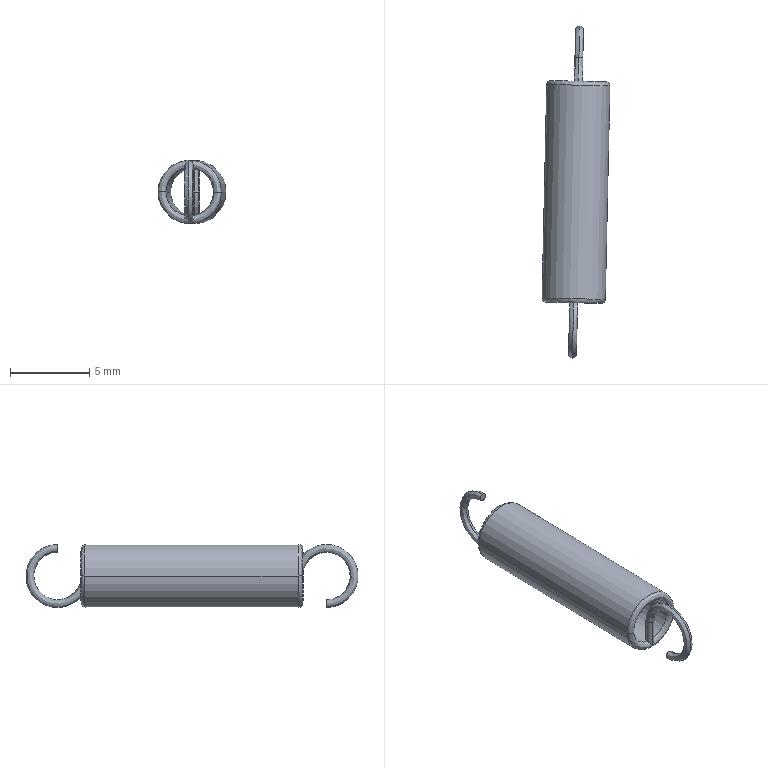Component | SolidWorks | YAUS-D4-L20-1 | 1 solid | 18 faces | box 4.29 x 21 x 4 mm | volume 80 mm3 | spline 8 | cylinder 8 | plane 2 | commonest cylinder face diameters 0.5 x4 4 x2 3 x2
STEP:
#1=CARTESIAN_POINT('',(-2.297,-0.5365,1.426));
#2=VERTEX_POINT('',#1);
#3=CARTESIAN_POINT('',(-2.347,-0.5355,1.485));
#4=VERTEX_POINT('',#3);
#5=CARTESIAN_POINT('',(-2.287,-0.5368,1.485));
#6=DIRECTION('',(0.0216,0.9998,-0.));
#7=DIRECTION('',(0.9998,-0.0216,0.));
#8=AXIS2_PLACEMENT_3D('',#5,#6,#7);
#9=CIRCLE('',#8,0.05906);
#10=EDGE_CURVE('',#2,#4,#9,.T.);
#11=ORIENTED_EDGE('',*,*,#10,.T.);
#12=CARTESIAN_POINT('',(-2.366,-0.5351,1.485));
#13=VERTEX_POINT('',#12);
#14=CARTESIAN_POINT('',(-2.356,-0.5353,1.485));
#15=DIRECTION('',(-0.,0.,-1.));
#16=DIRECTION('',(-0.9998,0.0216,0.));
#17=AXIS2_PLACEMENT_3D('',#14,#15,#16);
#18=CIRCLE('',#17,0.009843);
#19=EDGE_CURVE('',#4,#13,#18,.T.);
#20=ORIENTED_EDGE('',*,*,#19,.T.);
#21=CARTESIAN_POINT('',(-2.209,-0.5385,1.485));
#22=VERTEX_POINT('',#21);
#23=CARTESIAN_POINT('',(-2.287,-0.5368,1.485));
#24=DIRECTION('',(0.0216,0.9998,-0.));
#25=DIRECTION('',(-0.9998,0.0216,0.));
#26=AXIS2_PLACEMENT_3D('',#23,#24,#25);
#27=CIRCLE('',#26,0.07874);
#28=EDGE_CURVE('',#22,#13,#27,.T.);
#29=ORIENTED_EDGE('',*,*,#28,.F.);
#30=CARTESIAN_POINT('',(-2.228,-0.538,1.485));
#31=VERTEX_POINT('',#30);
#32=CARTESIAN_POINT('',(-2.219,-0.5382,1.485));
#33=DIRECTION('',(0.,0.,1.));
#34=DIRECTION('',(0.9998,-0.0216,0.));
#35=AXIS2_PLACEMENT_3D('',#32,#33,#34);
#36=CIRCLE('',#35,0.009843);
#37=EDGE_CURVE('',#31,#22,#36,.T.);
#38=ORIENTED_EDGE('',*,*,#37,.F.);
#39=CARTESIAN_POINT('',(-2.278,-0.537,1.426));
#40=VERTEX_POINT('',#39);
#41=CARTESIAN_POINT('',(-2.287,-0.5368,1.485));
#42=DIRECTION('',(0.0216,0.9998,-0.));
#43=DIRECTION('',(0.9998,-0.0216,0.));
#44=AXIS2_PLACEMENT_3D('',#41,#42,#43);
#45=CIRCLE('',#44,0.05906);
#46=EDGE_CURVE('',#31,#40,#45,.T.);
#47=ORIENTED_EDGE('',*,*,#46,.T.);
#48=CARTESIAN_POINT('',(-2.288,-0.5466,1.416));
#49=VERTEX_POINT('',#48);
#50=CARTESIAN_POINT('',(-2.278,-0.537,1.426));
#51=CARTESIAN_POINT('',(-2.278,-0.5377,1.426));
#52=CARTESIAN_POINT('',(-2.278,-0.5385,1.426));
#53=CARTESIAN_POINT('',(-2.278,-0.5396,1.426));
#54=CARTESIAN_POINT('',(-2.278,-0.5401,1.426));
#55=CARTESIAN_POINT('',(-2.278,-0.5407,1.425));
#56=CARTESIAN_POINT('',(-2.279,-0.541,1.425));
#57=CARTESIAN_POINT('',(-2.279,-0.5413,1.425));
#58=CARTESIAN_POINT('',(-2.279,-0.5419,1.425));
#59=CARTESIAN_POINT('',(-2.279,-0.5424,1.424));
#60=CARTESIAN_POINT('',(-2.28,-0.5432,1.424));
#61=CARTESIAN_POINT('',(-2.28,-0.5436,1.423));
#62=CARTESIAN_POINT('',(-2.281,-0.544,1.423));
#63=CARTESIAN_POINT('',(-2.281,-0.5442,1.423));
#64=CARTESIAN_POINT('',(-2.281,-0.5443,1.422));
#65=CARTESIAN_POINT('',(-2.281,-0.5444,1.422));
#66=CARTESIAN_POINT('',(-2.282,-0.5447,1.422));
#67=CARTESIAN_POINT('',(-2.282,-0.545,1.422));
#68=CARTESIAN_POINT('',(-2.283,-0.5454,1.421));
#69=CARTESIAN_POINT('',(-2.283,-0.5456,1.42));
#70=CARTESIAN_POINT('',(-2.284,-0.5459,1.42));
#71=CARTESIAN_POINT('',(-2.284,-0.546,1.419));
#72=CARTESIAN_POINT('',(-2.286,-0.5466,1.417));
#73=CARTESIAN_POINT('',(-2.287,-0.5466,1.416));
#74=CARTESIAN_POINT('',(-2.288,-0.5466,1.416));
#75=B_SPLINE_CURVE_WITH_KNOTS('',3,(#50,#51,#52,#53,#54,#55,#56,#57,#58,#59,#60,#61,#62,#63,#64,#65,#66,#67,#68,#69,#70,#71,#72,#73,#74),.UNSPECIFIED.,.F.,.F.,(4,2,1,2,2,2,1,1,2,2,2,2,2,4),(0.,0.125,0.1875,0.2187,0.25,0.375,0.4375,0.4687,0.4844,0.5,0.625,0.6875,0.75,1.),.UNSPECIFIED.);
#76=EDGE_CURVE('',#40,#49,#75,.T.);
#77=ORIENTED_EDGE('',*,*,#76,.T.);
#78=CARTESIAN_POINT('',(-2.288,-0.5466,1.416));
#79=CARTESIAN_POINT('',(-2.288,-0.5466,1.416));
#80=CARTESIAN_POINT('',(-2.288,-0.5466,1.416));
#81=CARTESIAN_POINT('',(-2.289,-0.5464,1.417));
#82=CARTESIAN_POINT('',(-2.29,-0.5464,1.418));
#83=CARTESIAN_POINT('',(-2.29,-0.5462,1.418));
#84=CARTESIAN_POINT('',(-2.291,-0.5461,1.419));
#85=CARTESIAN_POINT('',(-2.292,-0.5457,1.42));
#86=CARTESIAN_POINT('',(-2.292,-0.5454,1.42));
#87=CARTESIAN_POINT('',(-2.293,-0.5449,1.421));
#88=CARTESIAN_POINT('',(-2.293,-0.5448,1.421));
#89=CARTESIAN_POINT('',(-2.294,-0.5445,1.422));
#90=CARTESIAN_POINT('',(-2.294,-0.5444,1.422));
#91=CARTESIAN_POINT('',(-2.294,-0.5443,1.422));
#92=CARTESIAN_POINT('',(-2.294,-0.5442,1.422));
#93=CARTESIAN_POINT('',(-2.294,-0.5442,1.422));
#94=CARTESIAN_POINT('',(-2.295,-0.5437,1.423));
#95=CARTESIAN_POINT('',(-2.295,-0.5431,1.423));
#96=CARTESIAN_POINT('',(-2.296,-0.5424,1.424));
#97=CARTESIAN_POINT('',(-2.296,-0.542,1.424));
#98=CARTESIAN_POINT('',(-2.296,-0.5416,1.425));
#99=CARTESIAN_POINT('',(-2.296,-0.5413,1.425));
#100=CARTESIAN_POINT('',(-2.296,-0.5412,1.425));
#101=CARTESIAN_POINT('',(-2.297,-0.5396,1.426));
#102=CARTESIAN_POINT('',(-2.297,-0.538,1.426));
#103=CARTESIAN_POINT('',(-2.297,-0.5365,1.426));
#104=B_SPLINE_CURVE_WITH_KNOTS('',3,(#78,#79,#80,#81,#82,#83,#84,#85,#86,#87,#88,#89,#90,#91,#92,#93,#94,#95,#96,#97,#98,#99,#100,#101,#102,#103),.UNSPECIFIED.,.F.,.F.,(4,2,2,2,2,2,1,2,2,2,1,2,2,4),(0.,0.125,0.1875,0.25,0.375,0.4375,0.4688,0.4844,0.5,0.625,0.6875,0.7188,0.75,1.),.UNSPECIFIED.);
#105=EDGE_CURVE('',#49,#2,#104,.T.);
#106=ORIENTED_EDGE('',*,*,#105,.T.);
#107=EDGE_LOOP('',(#11,#20,#29,#38,#47,#77,#106));
#108=FACE_OUTER_BOUND('',#107,.T.);
#109=CARTESIAN_POINT('',(-2.347,-0.5355,1.485));
#110=CARTESIAN_POINT('',(-2.347,-0.5355,1.366));
#111=CARTESIAN_POINT('',(-2.228,-0.538,1.366));
#112=CARTESIAN_POINT('',(-2.228,-0.538,1.485));
#113=CARTESIAN_POINT('',(-2.347,-0.5412,1.485));
#114=CARTESIAN_POINT('',(-2.347,-0.5412,1.366));
#115=CARTESIAN_POINT('',(-2.229,-0.5438,1.366));
#116=CARTESIAN_POINT('',(-2.229,-0.5438,1.485));
#117=CARTESIAN_POINT('',(-2.351,-0.5452,1.485));
#118=CARTESIAN_POINT('',(-2.351,-0.5452,1.358));
#119=CARTESIAN_POINT('',(-2.225,-0.548,1.358));
#120=CARTESIAN_POINT('',(-2.225,-0.548,1.485));
#121=CARTESIAN_POINT('',(-2.357,-0.5451,1.485));
#122=CARTESIAN_POINT('',(-2.357,-0.5451,1.347));
#123=CARTESIAN_POINT('',(-2.219,-0.5481,1.347));
#124=CARTESIAN_POINT('',(-2.219,-0.5481,1.485));
#125=CARTESIAN_POINT('',(-2.362,-0.545,1.485));
#126=CARTESIAN_POINT('',(-2.362,-0.545,1.335));
#127=CARTESIAN_POINT('',(-2.213,-0.5482,1.335));
#128=CARTESIAN_POINT('',(-2.213,-0.5482,1.485));
#129=CARTESIAN_POINT('',(-2.366,-0.5408,1.485));
#130=CARTESIAN_POINT('',(-2.366,-0.5408,1.327));
#131=CARTESIAN_POINT('',(-2.209,-0.5442,1.327));
#132=CARTESIAN_POINT('',(-2.209,-0.5442,1.485));
#133=CARTESIAN_POINT('',(-2.366,-0.5351,1.485));
#134=CARTESIAN_POINT('',(-2.366,-0.5351,1.327));
#135=CARTESIAN_POINT('',(-2.209,-0.5385,1.327));
#136=CARTESIAN_POINT('',(-2.209,-0.5385,1.485));
#137=(BOUNDED_SURFACE()B_SPLINE_SURFACE(3,3,((#109,#110,#111,#112),(#113,#114,#115,#116),(#117,#118,#119,#120),(#121,#122,#123,#124),(#125,#126,#127,#128),(#129,#130,#131,#132),(#133,#134,#135,#136)),.UNSPECIFIED.,.F.,.F.,.F.)B_SPLINE_SURFACE_WITH_KNOTS((4,3,4),(4,4),(0.,0.5,1.),(0.,1.),.UNSPECIFIED.)GEOMETRIC_REPRESENTATION_ITEM()RATIONAL_B_SPLINE_SURFACE(((1.,0.3333,0.3333,1.),(0.8047,0.2682,0.2682,0.8047),(0.8047,0.2682,0.2682,0.8047),(1.,0.3333,0.3333,1.),(0.8047,0.2682,0.2682,0.8047),(0.8047,0.2682,0.2682,0.8047),(1.,0.3333,0.3333,1.)))REPRESENTATION_ITEM('')SURFACE());
#138=ADVANCED_FACE('',(#108),#137,.T.);
#139=CARTESIAN_POINT('',(-2.355,-0.003688,1.485));
#140=VERTEX_POINT('',#139);
#141=CARTESIAN_POINT('',(-2.197,-0.007089,1.485));
#142=VERTEX_POINT('',#141);
#143=CARTESIAN_POINT('',(-2.276,-0.005388,1.485));
#144=DIRECTION('',(-0.0216,-0.9998,0.));
#145=DIRECTION('',(-0.9998,0.0216,0.));
#146=AXIS2_PLACEMENT_3D('',#143,#144,#145);
#147=CIRCLE('',#146,0.07874);
#148=EDGE_CURVE('',#140,#142,#147,.T.);
#149=ORIENTED_EDGE('',*,*,#148,.F.);
#150=CARTESIAN_POINT('',(-2.335,-0.004113,1.485));
#151=VERTEX_POINT('',#150);
#152=CARTESIAN_POINT('',(-2.345,-0.003901,1.485));
#153=DIRECTION('',(-0.,0.,-1.));
#154=DIRECTION('',(-0.9998,0.0216,0.));
#155=AXIS2_PLACEMENT_3D('',#152,#153,#154);
#156=CIRCLE('',#155,0.009843);
#157=EDGE_CURVE('',#140,#151,#156,.T.);
#158=ORIENTED_EDGE('',*,*,#157,.T.);
#159=CARTESIAN_POINT('',(-2.217,-0.006664,1.485));
#160=VERTEX_POINT('',#159);
#161=CARTESIAN_POINT('',(-2.276,-0.005388,1.485));
#162=DIRECTION('',(-0.0216,-0.9998,0.));
#163=DIRECTION('',(0.9998,-0.0216,0.));
#164=AXIS2_PLACEMENT_3D('',#161,#162,#163);
#165=CIRCLE('',#164,0.05906);
#166=EDGE_CURVE('',#151,#160,#165,.T.);
#167=ORIENTED_EDGE('',*,*,#166,.T.);
#168=CARTESIAN_POINT('',(-2.207,-0.006876,1.485));
#169=DIRECTION('',(0.,0.,1.));
#170=DIRECTION('',(0.9998,-0.0216,0.));
#171=AXIS2_PLACEMENT_3D('',#168,#169,#170);
#172=CIRCLE('',#171,0.009843);
#173=EDGE_CURVE('',#142,#160,#172,.T.);
#174=ORIENTED_EDGE('',*,*,#173,.F.);
#175=EDGE_LOOP('',(#149,#158,#167,#174));
#176=FACE_OUTER_BOUND('',#175,.T.);
#177=CARTESIAN_POINT('',(-2.355,-0.003688,1.485));
#178=CARTESIAN_POINT('',(-2.355,-0.003688,1.327));
#179=CARTESIAN_POINT('',(-2.197,-0.007089,1.327));
#180=CARTESIAN_POINT('',(-2.197,-0.007089,1.485));
#181=CARTESIAN_POINT('',(-2.354,0.01599,1.485));
#182=CARTESIAN_POINT('',(-2.354,0.01599,1.327));
#183=CARTESIAN_POINT('',(-2.197,0.01259,1.327));
#184=CARTESIAN_POINT('',(-2.197,0.01259,1.485));
#185=CARTESIAN_POINT('',(-2.335,0.01557,1.485));
#186=CARTESIAN_POINT('',(-2.335,0.01557,1.366));
#187=CARTESIAN_POINT('',(-2.217,0.01302,1.366));
#188=CARTESIAN_POINT('',(-2.217,0.01302,1.485));
#189=CARTESIAN_POINT('',(-2.335,-0.004113,1.485));
#190=CARTESIAN_POINT('',(-2.335,-0.004113,1.366));
#191=CARTESIAN_POINT('',(-2.217,-0.006664,1.366));
#192=CARTESIAN_POINT('',(-2.217,-0.006664,1.485));
#193=(BOUNDED_SURFACE()B_SPLINE_SURFACE(3,3,((#177,#178,#179,#180),(#181,#182,#183,#184),(#185,#186,#187,#188),(#189,#190,#191,#192)),.UNSPECIFIED.,.F.,.F.,.F.)B_SPLINE_SURFACE_WITH_KNOTS((4,4),(4,4),(0.,1.),(0.,1.),.UNSPECIFIED.)GEOMETRIC_REPRESENTATION_ITEM()RATIONAL_B_SPLINE_SURFACE(((1.,0.3333,0.3333,1.),(0.3333,0.1111,0.1111,0.3333),(0.3333,0.1111,0.1111,0.3333),(1.,0.3333,0.3333,1.)))REPRESENTATION_ITEM('')SURFACE());
#194=ADVANCED_FACE('',(#176),#193,.T.);
#195=CARTESIAN_POINT('',(-2.287,-0.5368,1.485));
#196=DIRECTION('',(0.0216,0.9998,-0.));
#197=DIRECTION('',(-0.9998,0.0216,0.));
#198=AXIS2_PLACEMENT_3D('',#195,#196,#197);
#199=CIRCLE('',#198,0.07874);
#200=EDGE_CURVE('',#13,#22,#199,.T.);
#201=ORIENTED_EDGE('',*,*,#200,.T.);
#202=CARTESIAN_POINT('',(-2.209,-0.5483,1.485));
#203=DIRECTION('',(0.0216,0.9998,-0.));
#204=VECTOR('',#203,39.37);
#205=LINE('',#202,#204);
#206=EDGE_CURVE('',#22,#142,#205,.T.);
#207=ORIENTED_EDGE('',*,*,#206,.T.);
#208=CARTESIAN_POINT('',(-2.276,-0.005388,1.485));
#209=DIRECTION('',(-0.0216,-0.9998,0.));
#210=DIRECTION('',(-0.9998,0.0216,0.));
#211=AXIS2_PLACEMENT_3D('',#208,#209,#210);
#212=CIRCLE('',#211,0.07874);
#213=EDGE_CURVE('',#142,#140,#212,.T.);
#214=ORIENTED_EDGE('',*,*,#213,.T.);
#215=CARTESIAN_POINT('',(-2.366,-0.5449,1.485));
#216=DIRECTION('',(0.0216,0.9998,-0.));
#217=VECTOR('',#216,39.37);
#218=LINE('',#215,#217);
#219=EDGE_CURVE('',#13,#140,#218,.T.);
#220=ORIENTED_EDGE('',*,*,#219,.F.);
#221=EDGE_LOOP('',(#201,#207,#214,#220));
#222=FACE_OUTER_BOUND('',#221,.T.);
#223=CARTESIAN_POINT('',(-2.288,-0.5466,1.485));
#224=DIRECTION('',(0.0216,0.9998,-0.));
#225=DIRECTION('',(-0.9998,0.0216,0.));
#226=AXIS2_PLACEMENT_3D('',#223,#224,#225);
#227=CYLINDRICAL_SURFACE('',#226,0.07874);
#228=ADVANCED_FACE('',(#222),#227,.T.);
#229=ORIENTED_EDGE('',*,*,#105,.F.);
#230=CARTESIAN_POINT('',(-2.288,-0.5466,1.485));
#231=VERTEX_POINT('',#230);
#232=CARTESIAN_POINT('',(-2.288,-0.5466,1.416));
#233=DIRECTION('',(0.,0.,1.));
#234=VECTOR('',#233,39.37);
#235=LINE('',#232,#234);
#236=EDGE_CURVE('',#49,#231,#235,.T.);
#237=ORIENTED_EDGE('',*,*,#236,.T.);
#238=CARTESIAN_POINT('',(-2.287,-0.5269,1.485));
#239=VERTEX_POINT('',#238);
#240=CARTESIAN_POINT('',(-2.287,-0.5368,1.485));
#241=DIRECTION('',(-0.,-0.,-1.));
#242=DIRECTION('',(0.0216,0.9998,0.));
#243=AXIS2_PLACEMENT_3D('',#240,#241,#242);
#244=CIRCLE('',#243,0.009843);
#245=EDGE_CURVE('',#231,#239,#244,.T.);
#246=ORIENTED_EDGE('',*,*,#245,.T.);
#247=CARTESIAN_POINT('',(-2.287,-0.5269,1.426));
#248=VERTEX_POINT('',#247);
#249=CARTESIAN_POINT('',(-2.287,-0.5269,1.416));
#250=DIRECTION('',(0.,0.,1.));
#251=VECTOR('',#250,39.37);
#252=LINE('',#249,#251);
#253=EDGE_CURVE('',#248,#239,#252,.T.);
#254=ORIENTED_EDGE('',*,*,#253,.F.);
#255=CARTESIAN_POINT('',(-2.287,-0.5269,1.426));
#256=CARTESIAN_POINT('',(-2.29,-0.5269,1.426));
#257=CARTESIAN_POINT('',(-2.292,-0.5279,1.426));
#258=CARTESIAN_POINT('',(-2.296,-0.5314,1.426));
#259=CARTESIAN_POINT('',(-2.297,-0.5339,1.426));
#260=CARTESIAN_POINT('',(-2.297,-0.5365,1.426));
#261=B_SPLINE_CURVE_WITH_KNOTS('',3,(#255,#256,#257,#258,#259,#260),.UNSPECIFIED.,.F.,.F.,(4,2,4),(0.0003916,0.0005872,0.0007828),.UNSPECIFIED.);
#262=EDGE_CURVE('',#248,#2,#261,.T.);
#263=ORIENTED_EDGE('',*,*,#262,.T.);
#264=EDGE_LOOP('',(#229,#237,#246,#254,#263));
#265=FACE_OUTER_BOUND('',#264,.T.);
#266=CARTESIAN_POINT('',(-2.287,-0.5368,1.416));
#267=DIRECTION('',(0.,0.,1.));
#268=DIRECTION('',(0.0216,0.9998,0.));
#269=AXIS2_PLACEMENT_3D('',#266,#267,#268);
#270=CYLINDRICAL_SURFACE('',#269,0.009843);
#271=ADVANCED_FACE('',(#265),#270,.T.);
#272=ORIENTED_EDGE('',*,*,#46,.F.);
#273=CARTESIAN_POINT('',(-2.229,-0.5479,1.485));
#274=DIRECTION('',(0.0216,0.9998,-0.));
#275=VECTOR('',#274,39.37);
#276=LINE('',#273,#275);
#277=EDGE_CURVE('',#31,#160,#276,.T.);
#278=ORIENTED_EDGE('',*,*,#277,.T.);
#279=ORIENTED_EDGE('',*,*,#166,.F.);
#280=CARTESIAN_POINT('',(-2.347,-0.5453,1.485));
#281=DIRECTION('',(0.0216,0.9998,-0.));
#282=VECTOR('',#281,39.37);
#283=LINE('',#280,#282);
#284=EDGE_CURVE('',#4,#151,#283,.T.);
#285=ORIENTED_EDGE('',*,*,#284,.F.);
#286=ORIENTED_EDGE('',*,*,#10,.F.);
#287=ORIENTED_EDGE('',*,*,#262,.F.);
#288=CARTESIAN_POINT('',(-2.278,-0.537,1.426));
#289=CARTESIAN_POINT('',(-2.278,-0.5344,1.426));
#290=CARTESIAN_POINT('',(-2.279,-0.5318,1.426));
#291=CARTESIAN_POINT('',(-2.282,-0.5281,1.426));
#292=CARTESIAN_POINT('',(-2.285,-0.527,1.426));
#293=CARTESIAN_POINT('',(-2.287,-0.5269,1.426));
#294=B_SPLINE_CURVE_WITH_KNOTS('',3,(#288,#289,#290,#291,#292,#293),.UNSPECIFIED.,.F.,.F.,(4,2,4),(0.,0.0001958,0.0003916),.UNSPECIFIED.);
#295=EDGE_CURVE('',#40,#248,#294,.T.);
#296=ORIENTED_EDGE('',*,*,#295,.F.);
#297=EDGE_LOOP('',(#272,#278,#279,#285,#286,#287,#296));
#298=FACE_OUTER_BOUND('',#297,.T.);
#299=CARTESIAN_POINT('',(-2.288,-0.5466,1.485));
#300=DIRECTION('',(0.0216,0.9998,-0.));
#301=DIRECTION('',(-0.9998,0.0216,0.));
#302=AXIS2_PLACEMENT_3D('',#299,#300,#301);
#303=CYLINDRICAL_SURFACE('',#302,0.05906);
#304=ADVANCED_FACE('',(#298),#303,.F.);
#305=CARTESIAN_POINT('',(-2.276,0.004452,1.485));
#306=VERTEX_POINT('',#305);
#307=CARTESIAN_POINT('',(-2.276,-0.01523,1.485));
#308=VERTEX_POINT('',#307);
#309=CARTESIAN_POINT('',(-2.276,-0.005388,1.485));
#310=DIRECTION('',(0.,0.,1.));
#311=DIRECTION('',(0.0216,0.9998,0.));
#312=AXIS2_PLACEMENT_3D('',#309,#310,#311);
#313=CIRCLE('',#312,0.009843);
#314=EDGE_CURVE('',#306,#308,#313,.T.);
#315=ORIENTED_EDGE('',*,*,#314,.T.);
#316=CARTESIAN_POINT('',(-2.276,-0.01523,1.544));
#317=VERTEX_POINT('',#316);
#318=CARTESIAN_POINT('',(-2.276,-0.01523,1.485));
#319=DIRECTION('',(0.,0.,1.));
#320=VECTOR('',#319,39.37);
#321=LINE('',#318,#320);
#322=EDGE_CURVE('',#308,#317,#321,.T.);
#323=ORIENTED_EDGE('',*,*,#322,.T.);
#324=CARTESIAN_POINT('',(-2.286,-0.005176,1.543));
#325=VERTEX_POINT('',#324);
#326=CARTESIAN_POINT('',(-2.276,-0.01523,1.544));
#327=CARTESIAN_POINT('',(-2.279,-0.01517,1.544));
#328=CARTESIAN_POINT('',(-2.281,-0.01407,1.543));
#329=CARTESIAN_POINT('',(-2.285,-0.01033,1.543));
#330=CARTESIAN_POINT('',(-2.286,-0.00778,1.543));
#331=CARTESIAN_POINT('',(-2.286,-0.005176,1.543));
#332=B_SPLINE_CURVE_WITH_KNOTS('',3,(#326,#327,#328,#329,#330,#331),.UNSPECIFIED.,.F.,.F.,(4,2,4),(0.0003916,0.0005872,0.0007828),.UNSPECIFIED.);
#333=EDGE_CURVE('',#317,#325,#332,.T.);
#334=ORIENTED_EDGE('',*,*,#333,.T.);
#335=CARTESIAN_POINT('',(-2.276,0.004452,1.553));
#336=VERTEX_POINT('',#335);
#337=CARTESIAN_POINT('',(-2.276,0.004452,1.553));
#338=CARTESIAN_POINT('',(-2.276,0.004458,1.553));
#339=CARTESIAN_POINT('',(-2.277,0.004456,1.553));
#340=CARTESIAN_POINT('',(-2.277,0.004363,1.552));
#341=CARTESIAN_POINT('',(-2.278,0.004316,1.552));
#342=CARTESIAN_POINT('',(-2.278,0.004174,1.551));
#343=CARTESIAN_POINT('',(-2.279,0.004064,1.55));
#344=CARTESIAN_POINT('',(-2.28,0.003716,1.549));
#345=CARTESIAN_POINT('',(-2.28,0.00343,1.549));
#346=CARTESIAN_POINT('',(-2.281,0.002992,1.548));
#347=CARTESIAN_POINT('',(-2.281,0.002844,1.548));
#348=CARTESIAN_POINT('',(-2.282,0.002625,1.547));
#349=CARTESIAN_POINT('',(-2.282,0.002517,1.547));
#350=CARTESIAN_POINT('',(-2.282,0.002411,1.547));
#351=CARTESIAN_POINT('',(-2.282,0.002342,1.547));
#352=CARTESIAN_POINT('',(-2.282,0.00233,1.547));
#353=CARTESIAN_POINT('',(-2.283,0.001815,1.546));
#354=CARTESIAN_POINT('',(-2.283,0.001318,1.546));
#355=CARTESIAN_POINT('',(-2.284,0.0005523,1.545));
#356=CARTESIAN_POINT('',(-2.284,0.0001645,1.545));
#357=CARTESIAN_POINT('',(-2.284,-0.0002247,1.544));
#358=CARTESIAN_POINT('',(-2.285,-0.0004838,1.544));
#359=CARTESIAN_POINT('',(-2.285,-0.0005657,1.544));
#360=CARTESIAN_POINT('',(-2.285,-0.002154,1.543));
#361=CARTESIAN_POINT('',(-2.286,-0.003694,1.543));
#362=CARTESIAN_POINT('',(-2.286,-0.005176,1.543));
#363=B_SPLINE_CURVE_WITH_KNOTS('',3,(#337,#338,#339,#340,#341,#342,#343,#344,#345,#346,#347,#348,#349,#350,#351,#352,#353,#354,#355,#356,#357,#358,#359,#360,#361,#362),.UNSPECIFIED.,.F.,.F.,(4,2,2,2,2,2,1,2,2,2,1,2,2,4),(0.,0.125,0.1875,0.25,0.375,0.4375,0.4687,0.4844,0.5,0.625,0.6875,0.7188,0.75,1.),.UNSPECIFIED.);
#364=EDGE_CURVE('',#336,#325,#363,.T.);
#365=ORIENTED_EDGE('',*,*,#364,.F.);
#366=CARTESIAN_POINT('',(-2.276,0.004452,1.485));
#367=DIRECTION('',(0.,0.,1.));
#368=VECTOR('',#367,39.37);
#369=LINE('',#366,#368);
#370=EDGE_CURVE('',#306,#336,#369,.T.);
#371=ORIENTED_EDGE('',*,*,#370,.F.);
#372=EDGE_LOOP('',(#315,#323,#334,#365,#371));
#373=FACE_OUTER_BOUND('',#372,.T.);
#374=CARTESIAN_POINT('',(-2.276,-0.005388,1.485));
#375=DIRECTION('',(0.,0.,1.));
#376=DIRECTION('',(0.0216,0.9998,0.));
#377=AXIS2_PLACEMENT_3D('',#374,#375,#376);
#378=CYLINDRICAL_SURFACE('',#377,0.009843);
#379=ADVANCED_FACE('',(#373),#378,.T.);
#380=ORIENTED_EDGE('',*,*,#245,.F.);
#381=CARTESIAN_POINT('',(-2.289,-0.6056,1.426));
#382=VERTEX_POINT('',#381);
#383=CARTESIAN_POINT('',(-2.289,-0.6056,1.485));
#384=DIRECTION('',(0.9998,-0.0216,-0.));
#385=DIRECTION('',(0.0216,0.9998,0.));
#386=AXIS2_PLACEMENT_3D('',#383,#384,#385);
#387=CIRCLE('',#386,0.05906);
#388=EDGE_CURVE('',#231,#382,#387,.T.);
#389=ORIENTED_EDGE('',*,*,#388,.T.);
#390=CARTESIAN_POINT('',(-2.289,-0.6056,1.406));
#391=VERTEX_POINT('',#390);
#392=CARTESIAN_POINT('',(-2.289,-0.6056,1.426));
#393=CARTESIAN_POINT('',(-2.292,-0.6056,1.426));
#394=CARTESIAN_POINT('',(-2.294,-0.6055,1.424));
#395=CARTESIAN_POINT('',(-2.298,-0.6055,1.421));
#396=CARTESIAN_POINT('',(-2.299,-0.6054,1.418));
#397=CARTESIAN_POINT('',(-2.299,-0.6054,1.413));
#398=CARTESIAN_POINT('',(-2.298,-0.6055,1.411));
#399=CARTESIAN_POINT('',(-2.294,-0.6055,1.407));
#400=CARTESIAN_POINT('',(-2.292,-0.6056,1.406));
#401=CARTESIAN_POINT('',(-2.289,-0.6056,1.406));
#402=B_SPLINE_CURVE_WITH_KNOTS('',3,(#392,#393,#394,#395,#396,#397,#398,#399,#400,#401),.UNSPECIFIED.,.F.,.F.,(4,2,2,2,4),(0.001173,0.001368,0.001563,0.001759,0.001954),.UNSPECIFIED.);
#403=EDGE_CURVE('',#382,#391,#402,.T.);
#404=ORIENTED_EDGE('',*,*,#403,.T.);
#405=CARTESIAN_POINT('',(-2.289,-0.6056,1.485));
#406=DIRECTION('',(0.9998,-0.0216,-0.));
#407=DIRECTION('',(0.0216,0.9998,0.));
#408=AXIS2_PLACEMENT_3D('',#405,#406,#407);
#409=CIRCLE('',#408,0.07874);
#410=EDGE_CURVE('',#239,#391,#409,.T.);
#411=ORIENTED_EDGE('',*,*,#410,.F.);
#412=EDGE_LOOP('',(#380,#389,#404,#411));
#413=FACE_OUTER_BOUND('',#412,.T.);
#414=CARTESIAN_POINT('',(-2.287,-0.5269,1.485));
#415=CARTESIAN_POINT('',(-2.287,-0.5269,1.567));
#416=CARTESIAN_POINT('',(-2.289,-0.603,1.599));
#417=CARTESIAN_POINT('',(-2.29,-0.6613,1.54));
#418=CARTESIAN_POINT('',(-2.291,-0.7196,1.482));
#419=CARTESIAN_POINT('',(-2.291,-0.688,1.406));
#420=CARTESIAN_POINT('',(-2.289,-0.6056,1.406));
#421=CARTESIAN_POINT('',(-2.307,-0.5265,1.485));
#422=CARTESIAN_POINT('',(-2.307,-0.5265,1.567));
#423=CARTESIAN_POINT('',(-2.309,-0.6026,1.599));
#424=CARTESIAN_POINT('',(-2.31,-0.6609,1.54));
#425=CARTESIAN_POINT('',(-2.311,-0.7191,1.482));
#426=CARTESIAN_POINT('',(-2.31,-0.6876,1.406));
#427=CARTESIAN_POINT('',(-2.309,-0.6052,1.406));
#428=CARTESIAN_POINT('',(-2.307,-0.5462,1.485));
#429=CARTESIAN_POINT('',(-2.307,-0.5462,1.546));
#430=CARTESIAN_POINT('',(-2.309,-0.6033,1.57));
#431=CARTESIAN_POINT('',(-2.31,-0.647,1.526));
#432=CARTESIAN_POINT('',(-2.31,-0.6907,1.483));
#433=CARTESIAN_POINT('',(-2.31,-0.667,1.426));
#434=CARTESIAN_POINT('',(-2.309,-0.6052,1.426));
#435=CARTESIAN_POINT('',(-2.288,-0.5466,1.485));
#436=CARTESIAN_POINT('',(-2.288,-0.5466,1.546));
#437=CARTESIAN_POINT('',(-2.289,-0.6037,1.57));
#438=CARTESIAN_POINT('',(-2.29,-0.6474,1.526));
#439=CARTESIAN_POINT('',(-2.291,-0.6911,1.483));
#440=CARTESIAN_POINT('',(-2.29,-0.6674,1.426));
#441=CARTESIAN_POINT('',(-2.289,-0.6056,1.426));
#442=(BOUNDED_SURFACE()B_SPLINE_SURFACE(3,3,((#414,#415,#416,#417,#418,#419,#420),(#421,#422,#423,#424,#425,#426,#427),(#428,#429,#430,#431,#432,#433,#434),(#435,#436,#437,#438,#439,#440,#441)),.UNSPECIFIED.,.F.,.F.,.F.)B_SPLINE_SURFACE_WITH_KNOTS((4,4),(4,3,4),(0.,1.),(0.,0.5,1.),.UNSPECIFIED.)GEOMETRIC_REPRESENTATION_ITEM()RATIONAL_B_SPLINE_SURFACE(((1.,0.5885,0.5885,1.,0.5885,0.5885,1.),(0.3333,0.1962,0.1962,0.3333,0.1962,0.1962,0.3333),(0.3333,0.1962,0.1962,0.3333,0.1962,0.1962,0.3333),(1.,0.5885,0.5885,1.,0.5885,0.5885,1.)))REPRESENTATION_ITEM('')SURFACE());
#443=ADVANCED_FACE('',(#413),#442,.T.);
#444=CARTESIAN_POINT('',(-2.274,0.06349,1.563));
#445=VERTEX_POINT('',#444);
#446=CARTESIAN_POINT('',(-2.274,0.06349,1.544));
#447=VERTEX_POINT('',#446);
#448=CARTESIAN_POINT('',(-2.274,0.06349,1.563));
#449=CARTESIAN_POINT('',(-2.272,0.06344,1.563));
#450=CARTESIAN_POINT('',(-2.269,0.06338,1.562));
#451=CARTESIAN_POINT('',(-2.266,0.0633,1.559));
#452=CARTESIAN_POINT('',(-2.265,0.06328,1.556));
#453=CARTESIAN_POINT('',(-2.265,0.06328,1.551));
#454=CARTESIAN_POINT('',(-2.266,0.0633,1.548));
#455=CARTESIAN_POINT('',(-2.269,0.06338,1.545));
#456=CARTESIAN_POINT('',(-2.272,0.06344,1.544));
#457=CARTESIAN_POINT('',(-2.274,0.06349,1.544));
#458=B_SPLINE_CURVE_WITH_KNOTS('',3,(#448,#449,#450,#451,#452,#453,#454,#455,#456,#457),.UNSPECIFIED.,.F.,.F.,(4,2,2,2,4),(0.0003909,0.0005863,0.0007817,0.0009771,0.001173),.UNSPECIFIED.);
#459=EDGE_CURVE('',#445,#447,#458,.T.);
#460=ORIENTED_EDGE('',*,*,#459,.T.);
#461=CARTESIAN_POINT('',(-2.274,0.06349,1.485));
#462=DIRECTION('',(-0.9998,0.0216,0.));
#463=DIRECTION('',(-0.0216,-0.9998,0.));
#464=AXIS2_PLACEMENT_3D('',#461,#462,#463);
#465=CIRCLE('',#464,0.05906);
#466=EDGE_CURVE('',#447,#306,#465,.T.);
#467=ORIENTED_EDGE('',*,*,#466,.T.);
#468=CARTESIAN_POINT('',(-2.276,-0.005388,1.485));
#469=DIRECTION('',(0.,0.,1.));
#470=DIRECTION('',(0.0216,0.9998,0.));
#471=AXIS2_PLACEMENT_3D('',#468,#469,#470);
#472=CIRCLE('',#471,0.009843);
#473=EDGE_CURVE('',#308,#306,#472,.T.);
#474=ORIENTED_EDGE('',*,*,#473,.F.);
#475=CARTESIAN_POINT('',(-2.274,0.06349,1.485));
#476=DIRECTION('',(-0.9998,0.0216,0.));
#477=DIRECTION('',(-0.0216,-0.9998,0.));
#478=AXIS2_PLACEMENT_3D('',#475,#476,#477);
#479=CIRCLE('',#478,0.07874);
#480=EDGE_CURVE('',#445,#308,#479,.T.);
#481=ORIENTED_EDGE('',*,*,#480,.F.);
#482=EDGE_LOOP('',(#460,#467,#474,#481));
#483=FACE_OUTER_BOUND('',#482,.T.);
#484=CARTESIAN_POINT('',(-2.274,0.06349,1.563));
#485=CARTESIAN_POINT('',(-2.273,0.1459,1.563));
#486=CARTESIAN_POINT('',(-2.272,0.1774,1.487));
#487=CARTESIAN_POINT('',(-2.273,0.1192,1.429));
#488=CARTESIAN_POINT('',(-2.275,0.0609,1.371));
#489=CARTESIAN_POINT('',(-2.276,-0.01523,1.402));
#490=CARTESIAN_POINT('',(-2.276,-0.01523,1.485));
#491=CARTESIAN_POINT('',(-2.255,0.06307,1.563));
#492=CARTESIAN_POINT('',(-2.253,0.1455,1.563));
#493=CARTESIAN_POINT('',(-2.252,0.177,1.487));
#494=CARTESIAN_POINT('',(-2.254,0.1187,1.429));
#495=CARTESIAN_POINT('',(-2.255,0.06047,1.371));
#496=CARTESIAN_POINT('',(-2.257,-0.01565,1.402));
#497=CARTESIAN_POINT('',(-2.257,-0.01565,1.485));
#498=CARTESIAN_POINT('',(-2.255,0.06307,1.544));
#499=CARTESIAN_POINT('',(-2.253,0.1249,1.544));
#500=CARTESIAN_POINT('',(-2.253,0.1485,1.487));
#501=CARTESIAN_POINT('',(-2.254,0.1048,1.443));
#502=CARTESIAN_POINT('',(-2.255,0.06112,1.399));
#503=CARTESIAN_POINT('',(-2.256,0.004027,1.423));
#504=CARTESIAN_POINT('',(-2.256,0.004027,1.485));
#505=CARTESIAN_POINT('',(-2.274,0.06349,1.544));
#506=CARTESIAN_POINT('',(-2.273,0.1253,1.544));
#507=CARTESIAN_POINT('',(-2.273,0.1489,1.487));
#508=CARTESIAN_POINT('',(-2.274,0.1052,1.443));
#509=CARTESIAN_POINT('',(-2.275,0.06154,1.399));
#510=CARTESIAN_POINT('',(-2.276,0.004452,1.423));
#511=CARTESIAN_POINT('',(-2.276,0.004452,1.485));
#512=(BOUNDED_SURFACE()B_SPLINE_SURFACE(3,3,((#484,#485,#486,#487,#488,#489,#490),(#491,#492,#493,#494,#495,#496,#497),(#498,#499,#500,#501,#502,#503,#504),(#505,#506,#507,#508,#509,#510,#511)),.UNSPECIFIED.,.F.,.F.,.T.)B_SPLINE_SURFACE_WITH_KNOTS((4,4),(4,3,4),(0.,1.),(0.,0.5,1.),.UNSPECIFIED.)GEOMETRIC_REPRESENTATION_ITEM()RATIONAL_B_SPLINE_SURFACE(((1.,0.5885,0.5885,1.,0.5885,0.5885,1.),(0.3333,0.1962,0.1962,0.3333,0.1962,0.1962,0.3333),(0.3333,0.1962,0.1962,0.3333,0.1962,0.1962,0.3333),(1.,0.5885,0.5885,1.,0.5885,0.5885,1.)))REPRESENTATION_ITEM('')SURFACE());
#513=ADVANCED_FACE('',(#483),#512,.T.);
#514=ORIENTED_EDGE('',*,*,#206,.F.);
#515=ORIENTED_EDGE('',*,*,#28,.T.);
#516=ORIENTED_EDGE('',*,*,#219,.T.);
#517=ORIENTED_EDGE('',*,*,#148,.T.);
#518=EDGE_LOOP('',(#514,#515,#516,#517));
#519=FACE_OUTER_BOUND('',#518,.T.);
#520=CARTESIAN_POINT('',(-2.288,-0.5466,1.485));
#521=DIRECTION('',(0.0216,0.9998,-0.));
#522=DIRECTION('',(-0.9998,0.0216,0.));
#523=AXIS2_PLACEMENT_3D('',#520,#521,#522);
#524=CYLINDRICAL_SURFACE('',#523,0.07874);
#525=ADVANCED_FACE('',(#519),#524,.T.);
#526=ORIENTED_EDGE('',*,*,#19,.F.);
#527=CARTESIAN_POINT('',(-2.287,-0.5368,1.485));
#528=DIRECTION('',(0.0216,0.9998,-0.));
#529=DIRECTION('',(0.9998,-0.0216,0.));
#530=AXIS2_PLACEMENT_3D('',#527,#528,#529);
#531=CIRCLE('',#530,0.05906);
#532=EDGE_CURVE('',#4,#31,#531,.T.);
#533=ORIENTED_EDGE('',*,*,#532,.T.);
#534=ORIENTED_EDGE('',*,*,#37,.T.);
#535=ORIENTED_EDGE('',*,*,#200,.F.);
#536=EDGE_LOOP('',(#526,#533,#534,#535));
#537=FACE_OUTER_BOUND('',#536,.T.);
#538=CARTESIAN_POINT('',(-2.228,-0.538,1.485));
#539=CARTESIAN_POINT('',(-2.228,-0.538,1.603));
#540=CARTESIAN_POINT('',(-2.347,-0.5355,1.603));
#541=CARTESIAN_POINT('',(-2.347,-0.5355,1.485));
#542=CARTESIAN_POINT('',(-2.229,-0.5438,1.485));
#543=CARTESIAN_POINT('',(-2.229,-0.5438,1.603));
#544=CARTESIAN_POINT('',(-2.347,-0.5412,1.603));
#545=CARTESIAN_POINT('',(-2.347,-0.5412,1.485));
#546=CARTESIAN_POINT('',(-2.225,-0.548,1.485));
#547=CARTESIAN_POINT('',(-2.225,-0.548,1.611));
#548=CARTESIAN_POINT('',(-2.351,-0.5452,1.611));
#549=CARTESIAN_POINT('',(-2.351,-0.5452,1.485));
#550=CARTESIAN_POINT('',(-2.219,-0.5481,1.485));
#551=CARTESIAN_POINT('',(-2.219,-0.5481,1.622));
#552=CARTESIAN_POINT('',(-2.357,-0.5451,1.622));
#553=CARTESIAN_POINT('',(-2.357,-0.5451,1.485));
#554=CARTESIAN_POINT('',(-2.213,-0.5482,1.485));
#555=CARTESIAN_POINT('',(-2.213,-0.5482,1.634));
#556=CARTESIAN_POINT('',(-2.362,-0.545,1.634));
#557=CARTESIAN_POINT('',(-2.362,-0.545,1.485));
#558=CARTESIAN_POINT('',(-2.209,-0.5442,1.485));
#559=CARTESIAN_POINT('',(-2.209,-0.5442,1.642));
#560=CARTESIAN_POINT('',(-2.366,-0.5408,1.642));
#561=CARTESIAN_POINT('',(-2.366,-0.5408,1.485));
#562=CARTESIAN_POINT('',(-2.209,-0.5385,1.485));
#563=CARTESIAN_POINT('',(-2.209,-0.5385,1.642));
#564=CARTESIAN_POINT('',(-2.366,-0.5351,1.642));
#565=CARTESIAN_POINT('',(-2.366,-0.5351,1.485));
#566=(BOUNDED_SURFACE()B_SPLINE_SURFACE(3,3,((#538,#539,#540,#541),(#542,#543,#544,#545),(#546,#547,#548,#549),(#550,#551,#552,#553),(#554,#555,#556,#557),(#558,#559,#560,#561),(#562,#563,#564,#565)),.UNSPECIFIED.,.F.,.F.,.F.)B_SPLINE_SURFACE_WITH_KNOTS((4,3,4),(4,4),(0.,0.5,1.),(0.,1.),.UNSPECIFIED.)GEOMETRIC_REPRESENTATION_ITEM()RATIONAL_B_SPLINE_SURFACE(((1.,0.3333,0.3333,1.),(0.8047,0.2682,0.2682,0.8047),(0.8047,0.2682,0.2682,0.8047),(1.,0.3333,0.3333,1.),(0.8047,0.2682,0.2682,0.8047),(0.8047,0.2682,0.2682,0.8047),(1.,0.3333,0.3333,1.)))REPRESENTATION_ITEM('')SURFACE());
#567=ADVANCED_FACE('',(#537),#566,.T.);
#568=ORIENTED_EDGE('',*,*,#157,.F.);
#569=ORIENTED_EDGE('',*,*,#213,.F.);
#570=ORIENTED_EDGE('',*,*,#173,.T.);
#571=CARTESIAN_POINT('',(-2.266,-0.005601,1.543));
#572=VERTEX_POINT('',#571);
#573=CARTESIAN_POINT('',(-2.276,-0.005388,1.485));
#574=DIRECTION('',(-0.0216,-0.9998,0.));
#575=DIRECTION('',(0.9998,-0.0216,0.));
#576=AXIS2_PLACEMENT_3D('',#573,#574,#575);
#577=CIRCLE('',#576,0.05906);
#578=EDGE_CURVE('',#160,#572,#577,.T.);
#579=ORIENTED_EDGE('',*,*,#578,.T.);
#580=CARTESIAN_POINT('',(-2.266,-0.005601,1.543));
#581=CARTESIAN_POINT('',(-2.266,-0.004862,1.543));
#582=CARTESIAN_POINT('',(-2.266,-0.004106,1.543));
#583=CARTESIAN_POINT('',(-2.266,-0.002978,1.543));
#584=CARTESIAN_POINT('',(-2.267,-0.002415,1.543));
#585=CARTESIAN_POINT('',(-2.267,-0.001861,1.544));
#586=CARTESIAN_POINT('',(-2.267,-0.001495,1.544));
#587=CARTESIAN_POINT('',(-2.267,-0.001265,1.544));
#588=CARTESIAN_POINT('',(-2.267,-0.0006049,1.544));
#589=CARTESIAN_POINT('',(-2.268,-0.00006661,1.545));
#590=CARTESIAN_POINT('',(-2.268,0.0007263,1.545));
#591=CARTESIAN_POINT('',(-2.269,0.001119,1.546));
#592=CARTESIAN_POINT('',(-2.269,0.001562,1.546));
#593=CARTESIAN_POINT('',(-2.269,0.001748,1.546));
#594=CARTESIAN_POINT('',(-2.269,0.001871,1.547));
#595=CARTESIAN_POINT('',(-2.269,0.001956,1.547));
#596=CARTESIAN_POINT('',(-2.27,0.002284,1.547));
#597=CARTESIAN_POINT('',(-2.27,0.002602,1.548));
#598=CARTESIAN_POINT('',(-2.271,0.003074,1.548));
#599=CARTESIAN_POINT('',(-2.271,0.00323,1.549));
#600=CARTESIAN_POINT('',(-2.272,0.003529,1.549));
#601=CARTESIAN_POINT('',(-2.272,0.003655,1.55));
#602=CARTESIAN_POINT('',(-2.274,0.004397,1.552));
#603=CARTESIAN_POINT('',(-2.275,0.004439,1.553));
#604=CARTESIAN_POINT('',(-2.276,0.004452,1.553));
#605=B_SPLINE_CURVE_WITH_KNOTS('',3,(#580,#581,#582,#583,#584,#585,#586,#587,#588,#589,#590,#591,#592,#593,#594,#595,#596,#597,#598,#599,#600,#601,#602,#603,#604),.UNSPECIFIED.,.F.,.F.,(4,2,1,2,2,2,1,1,2,2,2,2,2,4),(0.,0.125,0.1875,0.2188,0.25,0.375,0.4375,0.4688,0.4844,0.5,0.625,0.6875,0.75,1.),.UNSPECIFIED.);
#606=EDGE_CURVE('',#572,#336,#605,.T.);
#607=ORIENTED_EDGE('',*,*,#606,.T.);
#608=ORIENTED_EDGE('',*,*,#364,.T.);
#609=CARTESIAN_POINT('',(-2.276,-0.005388,1.485));
#610=DIRECTION('',(-0.0216,-0.9998,0.));
#611=DIRECTION('',(0.9998,-0.0216,0.));
#612=AXIS2_PLACEMENT_3D('',#609,#610,#611);
#613=CIRCLE('',#612,0.05906);
#614=EDGE_CURVE('',#325,#151,#613,.T.);
#615=ORIENTED_EDGE('',*,*,#614,.T.);
#616=EDGE_LOOP('',(#568,#569,#570,#579,#607,#608,#615));
#617=FACE_OUTER_BOUND('',#616,.T.);
#618=CARTESIAN_POINT('',(-2.197,-0.007089,1.485));
#619=CARTESIAN_POINT('',(-2.197,-0.007089,1.642));
#620=CARTESIAN_POINT('',(-2.355,-0.003688,1.642));
#621=CARTESIAN_POINT('',(-2.355,-0.003688,1.485));
#622=CARTESIAN_POINT('',(-2.197,0.01259,1.485));
#623=CARTESIAN_POINT('',(-2.197,0.01259,1.642));
#624=CARTESIAN_POINT('',(-2.354,0.01599,1.642));
#625=CARTESIAN_POINT('',(-2.354,0.01599,1.485));
#626=CARTESIAN_POINT('',(-2.217,0.01302,1.485));
#627=CARTESIAN_POINT('',(-2.217,0.01302,1.603));
#628=CARTESIAN_POINT('',(-2.335,0.01557,1.603));
#629=CARTESIAN_POINT('',(-2.335,0.01557,1.485));
#630=CARTESIAN_POINT('',(-2.217,-0.006664,1.485));
#631=CARTESIAN_POINT('',(-2.217,-0.006664,1.603));
#632=CARTESIAN_POINT('',(-2.335,-0.004113,1.603));
#633=CARTESIAN_POINT('',(-2.335,-0.004113,1.485));
#634=(BOUNDED_SURFACE()B_SPLINE_SURFACE(3,3,((#618,#619,#620,#621),(#622,#623,#624,#625),(#626,#627,#628,#629),(#630,#631,#632,#633)),.UNSPECIFIED.,.F.,.F.,.T.)B_SPLINE_SURFACE_WITH_KNOTS((4,4),(4,4),(0.,1.),(0.,1.),.UNSPECIFIED.)GEOMETRIC_REPRESENTATION_ITEM()RATIONAL_B_SPLINE_SURFACE(((1.,0.3333,0.3333,1.),(0.3333,0.1111,0.1111,0.3333),(0.3333,0.1111,0.1111,0.3333),(1.,0.3333,0.3333,1.)))REPRESENTATION_ITEM('')SURFACE());
#635=ADVANCED_FACE('',(#617),#634,.T.);
#636=ORIENTED_EDGE('',*,*,#236,.F.);
#637=ORIENTED_EDGE('',*,*,#76,.F.);
#638=ORIENTED_EDGE('',*,*,#295,.T.);
#639=ORIENTED_EDGE('',*,*,#253,.T.);
#640=CARTESIAN_POINT('',(-2.287,-0.5368,1.485));
#641=DIRECTION('',(-0.,-0.,-1.));
#642=DIRECTION('',(0.0216,0.9998,0.));
#643=AXIS2_PLACEMENT_3D('',#640,#641,#642);
#644=CIRCLE('',#643,0.009843);
#645=EDGE_CURVE('',#239,#231,#644,.T.);
#646=ORIENTED_EDGE('',*,*,#645,.T.);
#647=EDGE_LOOP('',(#636,#637,#638,#639,#646));
#648=FACE_OUTER_BOUND('',#647,.T.);
#649=CARTESIAN_POINT('',(-2.287,-0.5368,1.416));
#650=DIRECTION('',(0.,0.,1.));
#651=DIRECTION('',(0.0216,0.9998,0.));
#652=AXIS2_PLACEMENT_3D('',#649,#650,#651);
#653=CYLINDRICAL_SURFACE('',#652,0.009843);
#654=ADVANCED_FACE('',(#648),#653,.T.);
#655=ORIENTED_EDGE('',*,*,#277,.F.);
#656=ORIENTED_EDGE('',*,*,#532,.F.);
#657=ORIENTED_EDGE('',*,*,#284,.T.);
#658=ORIENTED_EDGE('',*,*,#614,.F.);
#659=ORIENTED_EDGE('',*,*,#333,.F.);
#660=CARTESIAN_POINT('',(-2.266,-0.005601,1.543));
#661=CARTESIAN_POINT('',(-2.266,-0.008207,1.543));
#662=CARTESIAN_POINT('',(-2.267,-0.01073,1.543));
#663=CARTESIAN_POINT('',(-2.271,-0.01427,1.543));
#664=CARTESIAN_POINT('',(-2.274,-0.01528,1.544));
#665=CARTESIAN_POINT('',(-2.276,-0.01523,1.544));
#666=B_SPLINE_CURVE_WITH_KNOTS('',3,(#660,#661,#662,#663,#664,#665),.UNSPECIFIED.,.F.,.F.,(4,2,4),(0.,0.0001958,0.0003916),.UNSPECIFIED.);
#667=EDGE_CURVE('',#572,#317,#666,.T.);
#668=ORIENTED_EDGE('',*,*,#667,.F.);
#669=ORIENTED_EDGE('',*,*,#578,.F.);
#670=EDGE_LOOP('',(#655,#656,#657,#658,#659,#668,#669));
#671=FACE_OUTER_BOUND('',#670,.T.);
#672=CARTESIAN_POINT('',(-2.288,-0.5466,1.485));
#673=DIRECTION('',(0.0216,0.9998,-0.));
#674=DIRECTION('',(-0.9998,0.0216,0.));
#675=AXIS2_PLACEMENT_3D('',#672,#673,#674);
#676=CYLINDRICAL_SURFACE('',#675,0.05906);
#677=ADVANCED_FACE('',(#671),#676,.F.);
#678=ORIENTED_EDGE('',*,*,#322,.F.);
#679=ORIENTED_EDGE('',*,*,#473,.T.);
#680=ORIENTED_EDGE('',*,*,#370,.T.);
#681=ORIENTED_EDGE('',*,*,#606,.F.);
#682=ORIENTED_EDGE('',*,*,#667,.T.);
#683=EDGE_LOOP('',(#678,#679,#680,#681,#682));
#684=FACE_OUTER_BOUND('',#683,.T.);
#685=CARTESIAN_POINT('',(-2.276,-0.005388,1.485));
#686=DIRECTION('',(0.,0.,1.));
#687=DIRECTION('',(0.0216,0.9998,0.));
#688=AXIS2_PLACEMENT_3D('',#685,#686,#687);
#689=CYLINDRICAL_SURFACE('',#688,0.009843);
#690=ADVANCED_FACE('',(#684),#689,.T.);
#691=ORIENTED_EDGE('',*,*,#388,.F.);
#692=ORIENTED_EDGE('',*,*,#645,.F.);
#693=ORIENTED_EDGE('',*,*,#410,.T.);
#694=CARTESIAN_POINT('',(-2.289,-0.6056,1.406));
#695=CARTESIAN_POINT('',(-2.286,-0.6057,1.406));
#696=CARTESIAN_POINT('',(-2.284,-0.6058,1.407));
#697=CARTESIAN_POINT('',(-2.28,-0.6058,1.411));
#698=CARTESIAN_POINT('',(-2.279,-0.6059,1.413));
#699=CARTESIAN_POINT('',(-2.279,-0.6059,1.418));
#700=CARTESIAN_POINT('',(-2.28,-0.6058,1.421));
#701=CARTESIAN_POINT('',(-2.284,-0.6058,1.424));
#702=CARTESIAN_POINT('',(-2.286,-0.6057,1.426));
#703=CARTESIAN_POINT('',(-2.289,-0.6056,1.426));
#704=B_SPLINE_CURVE_WITH_KNOTS('',3,(#694,#695,#696,#697,#698,#699,#700,#701,#702,#703),.UNSPECIFIED.,.F.,.F.,(4,2,2,2,4),(0.0003909,0.0005863,0.0007817,0.0009771,0.001173),.UNSPECIFIED.);
#705=EDGE_CURVE('',#391,#382,#704,.T.);
#706=ORIENTED_EDGE('',*,*,#705,.T.);
#707=EDGE_LOOP('',(#691,#692,#693,#706));
#708=FACE_OUTER_BOUND('',#707,.T.);
#709=CARTESIAN_POINT('',(-2.288,-0.5466,1.485));
#710=CARTESIAN_POINT('',(-2.288,-0.5466,1.546));
#711=CARTESIAN_POINT('',(-2.289,-0.6037,1.57));
#712=CARTESIAN_POINT('',(-2.29,-0.6474,1.526));
#713=CARTESIAN_POINT('',(-2.291,-0.6911,1.483));
#714=CARTESIAN_POINT('',(-2.29,-0.6674,1.426));
#715=CARTESIAN_POINT('',(-2.289,-0.6056,1.426));
#716=CARTESIAN_POINT('',(-2.268,-0.547,1.485));
#717=CARTESIAN_POINT('',(-2.268,-0.547,1.546));
#718=CARTESIAN_POINT('',(-2.269,-0.6041,1.57));
#719=CARTESIAN_POINT('',(-2.27,-0.6478,1.526));
#720=CARTESIAN_POINT('',(-2.271,-0.6915,1.483));
#721=CARTESIAN_POINT('',(-2.271,-0.6679,1.426));
#722=CARTESIAN_POINT('',(-2.269,-0.6061,1.426));
#723=CARTESIAN_POINT('',(-2.268,-0.5273,1.485));
#724=CARTESIAN_POINT('',(-2.268,-0.5273,1.567));
#725=CARTESIAN_POINT('',(-2.269,-0.6035,1.599));
#726=CARTESIAN_POINT('',(-2.27,-0.6617,1.54));
#727=CARTESIAN_POINT('',(-2.272,-0.72,1.482));
#728=CARTESIAN_POINT('',(-2.271,-0.6885,1.406));
#729=CARTESIAN_POINT('',(-2.269,-0.6061,1.406));
#730=CARTESIAN_POINT('',(-2.287,-0.5269,1.485));
#731=CARTESIAN_POINT('',(-2.287,-0.5269,1.567));
#732=CARTESIAN_POINT('',(-2.289,-0.603,1.599));
#733=CARTESIAN_POINT('',(-2.29,-0.6613,1.54));
#734=CARTESIAN_POINT('',(-2.291,-0.7196,1.482));
#735=CARTESIAN_POINT('',(-2.291,-0.688,1.406));
#736=CARTESIAN_POINT('',(-2.289,-0.6056,1.406));
#737=(BOUNDED_SURFACE()B_SPLINE_SURFACE(3,3,((#709,#710,#711,#712,#713,#714,#715),(#716,#717,#718,#719,#720,#721,#722),(#723,#724,#725,#726,#727,#728,#729),(#730,#731,#732,#733,#734,#735,#736)),.UNSPECIFIED.,.F.,.F.,.F.)B_SPLINE_SURFACE_WITH_KNOTS((4,4),(4,3,4),(0.,1.),(0.,0.5,1.),.UNSPECIFIED.)GEOMETRIC_REPRESENTATION_ITEM()RATIONAL_B_SPLINE_SURFACE(((1.,0.5885,0.5885,1.,0.5885,0.5885,1.),(0.3333,0.1962,0.1962,0.3333,0.1962,0.1962,0.3333),(0.3333,0.1962,0.1962,0.3333,0.1962,0.1962,0.3333),(1.,0.5885,0.5885,1.,0.5885,0.5885,1.)))REPRESENTATION_ITEM('')SURFACE());
#738=ADVANCED_FACE('',(#708),#737,.T.);
#739=ORIENTED_EDGE('',*,*,#466,.F.);
#740=CARTESIAN_POINT('',(-2.274,0.06349,1.544));
#741=CARTESIAN_POINT('',(-2.277,0.06355,1.544));
#742=CARTESIAN_POINT('',(-2.28,0.0636,1.545));
#743=CARTESIAN_POINT('',(-2.283,0.06368,1.548));
#744=CARTESIAN_POINT('',(-2.284,0.06371,1.551));
#745=CARTESIAN_POINT('',(-2.284,0.06371,1.556));
#746=CARTESIAN_POINT('',(-2.283,0.06368,1.559));
#747=CARTESIAN_POINT('',(-2.28,0.0636,1.562));
#748=CARTESIAN_POINT('',(-2.277,0.06355,1.563));
#749=CARTESIAN_POINT('',(-2.274,0.06349,1.563));
#750=B_SPLINE_CURVE_WITH_KNOTS('',3,(#740,#741,#742,#743,#744,#745,#746,#747,#748,#749),.UNSPECIFIED.,.F.,.F.,(4,2,2,2,4),(0.001173,0.001368,0.001563,0.001759,0.001954),.UNSPECIFIED.);
#751=EDGE_CURVE('',#447,#445,#750,.T.);
#752=ORIENTED_EDGE('',*,*,#751,.T.);
#753=ORIENTED_EDGE('',*,*,#480,.T.);
#754=ORIENTED_EDGE('',*,*,#314,.F.);
#755=EDGE_LOOP('',(#739,#752,#753,#754));
#756=FACE_OUTER_BOUND('',#755,.T.);
#757=CARTESIAN_POINT('',(-2.274,0.06349,1.544));
#758=CARTESIAN_POINT('',(-2.273,0.1253,1.544));
#759=CARTESIAN_POINT('',(-2.273,0.1489,1.487));
#760=CARTESIAN_POINT('',(-2.274,0.1052,1.443));
#761=CARTESIAN_POINT('',(-2.275,0.06154,1.399));
#762=CARTESIAN_POINT('',(-2.276,0.004452,1.423));
#763=CARTESIAN_POINT('',(-2.276,0.004452,1.485));
#764=CARTESIAN_POINT('',(-2.294,0.06392,1.544));
#765=CARTESIAN_POINT('',(-2.293,0.1257,1.544));
#766=CARTESIAN_POINT('',(-2.292,0.1494,1.487));
#767=CARTESIAN_POINT('',(-2.293,0.1057,1.443));
#768=CARTESIAN_POINT('',(-2.294,0.06197,1.399));
#769=CARTESIAN_POINT('',(-2.295,0.004877,1.423));
#770=CARTESIAN_POINT('',(-2.295,0.004877,1.485));
#771=CARTESIAN_POINT('',(-2.294,0.06392,1.563));
#772=CARTESIAN_POINT('',(-2.292,0.1463,1.563));
#773=CARTESIAN_POINT('',(-2.292,0.1778,1.487));
#774=CARTESIAN_POINT('',(-2.293,0.1196,1.429));
#775=CARTESIAN_POINT('',(-2.294,0.06132,1.371));
#776=CARTESIAN_POINT('',(-2.296,-0.0148,1.402));
#777=CARTESIAN_POINT('',(-2.296,-0.0148,1.485));
#778=CARTESIAN_POINT('',(-2.274,0.06349,1.563));
#779=CARTESIAN_POINT('',(-2.273,0.1459,1.563));
#780=CARTESIAN_POINT('',(-2.272,0.1774,1.487));
#781=CARTESIAN_POINT('',(-2.273,0.1192,1.429));
#782=CARTESIAN_POINT('',(-2.275,0.0609,1.371));
#783=CARTESIAN_POINT('',(-2.276,-0.01523,1.402));
#784=CARTESIAN_POINT('',(-2.276,-0.01523,1.485));
#785=(BOUNDED_SURFACE()B_SPLINE_SURFACE(3,3,((#757,#758,#759,#760,#761,#762,#763),(#764,#765,#766,#767,#768,#769,#770),(#771,#772,#773,#774,#775,#776,#777),(#778,#779,#780,#781,#782,#783,#784)),.UNSPECIFIED.,.F.,.F.,.F.)B_SPLINE_SURFACE_WITH_KNOTS((4,4),(4,3,4),(0.,1.),(0.,0.5,1.),.UNSPECIFIED.)GEOMETRIC_REPRESENTATION_ITEM()RATIONAL_B_SPLINE_SURFACE(((1.,0.5885,0.5885,1.,0.5885,0.5885,1.),(0.3333,0.1962,0.1962,0.3333,0.1962,0.1962,0.3333),(0.3333,0.1962,0.1962,0.3333,0.1962,0.1962,0.3333),(1.,0.5885,0.5885,1.,0.5885,0.5885,1.)))REPRESENTATION_ITEM('')SURFACE());
#786=ADVANCED_FACE('',(#756),#785,.T.);
#787=ORIENTED_EDGE('',*,*,#705,.F.);
#788=ORIENTED_EDGE('',*,*,#403,.F.);
#789=EDGE_LOOP('',(#787,#788));
#790=FACE_OUTER_BOUND('',#789,.T.);
#791=CARTESIAN_POINT('',(-2.289,-0.6056,1.416));
#792=DIRECTION('',(0.0216,0.9998,-0.));
#793=DIRECTION('',(-0.,-0.,-1.));
#794=AXIS2_PLACEMENT_3D('',#791,#792,#793);
#795=PLANE('',#794);
#796=ADVANCED_FACE('',(#790),#795,.T.);
#797=ORIENTED_EDGE('',*,*,#459,.F.);
#798=ORIENTED_EDGE('',*,*,#751,.F.);
#799=EDGE_LOOP('',(#797,#798));
#800=FACE_OUTER_BOUND('',#799,.T.);
#801=CARTESIAN_POINT('',(-2.274,0.06349,1.553));
#802=DIRECTION('',(0.0216,0.9998,-0.));
#803=DIRECTION('',(-0.,-0.,-1.));
#804=AXIS2_PLACEMENT_3D('',#801,#802,#803);
#805=PLANE('',#804);
#806=ADVANCED_FACE('',(#800),#805,.F.);
#807=CLOSED_SHELL('',(#138,#194,#228,#271,#304,#379,#443,#513,#525,#567,#635,#654,#677,#690,#738,#786,#796,#806));
#808=MANIFOLD_SOLID_BREP('',#807);
#809=CARTESIAN_POINT('',(0.,0.,0.));
#810=DIRECTION('',(0.,0.,1.));
#811=DIRECTION('',(1.,0.,0.));
#812=AXIS2_PLACEMENT_3D('',#809,#810,#811);
#813=(LENGTH_UNIT()NAMED_UNIT(*)SI_UNIT($,.METRE.));
#814=LENGTH_MEASURE_WITH_UNIT(LENGTH_MEASURE(0.0254),#813);
#815=DIMENSIONAL_EXPONENTS(1.,0.,0.,0.,0.,0.,0.);
#816=(CONVERSION_BASED_UNIT('',#814)LENGTH_UNIT()NAMED_UNIT(#815));
#817=UNCERTAINTY_MEASURE_WITH_UNIT(LENGTH_MEASURE(0.00001),#816,'','');
#818=(NAMED_UNIT(*)PLANE_ANGLE_UNIT()SI_UNIT($,.RADIAN.));
#819=(NAMED_UNIT(*)SI_UNIT($,.STERADIAN.)SOLID_ANGLE_UNIT());
#820=(GEOMETRIC_REPRESENTATION_CONTEXT(3)GLOBAL_UNCERTAINTY_ASSIGNED_CONTEXT((#817))GLOBAL_UNIT_ASSIGNED_CONTEXT((#816,#818,#819))REPRESENTATION_CONTEXT('',''));
#821=ADVANCED_BREP_SHAPE_REPRESENTATION('',(#808,#812),#820);
#822=COLOUR_RGB('',0.7922,0.8196,0.9333);
#823=FILL_AREA_STYLE_COLOUR('',#822);
#824=FILL_AREA_STYLE('',(#823));
#825=SURFACE_STYLE_FILL_AREA(#824);
#826=SURFACE_SIDE_STYLE('',(#825));
#827=SURFACE_STYLE_USAGE(.BOTH.,#826);
#828=PRESENTATION_STYLE_ASSIGNMENT((#827));
#829=STYLED_ITEM('',(#828),#808);
#830=PRESENTATION_LAYER_ASSIGNMENT('','',(#829));
#831=(LENGTH_UNIT()NAMED_UNIT(*)SI_UNIT($,.METRE.));
#832=LENGTH_MEASURE_WITH_UNIT(LENGTH_MEASURE(0.0254),#831);
#833=DIMENSIONAL_EXPONENTS(1.,0.,0.,0.,0.,0.,0.);
#834=(CONVERSION_BASED_UNIT('',#832)LENGTH_UNIT()NAMED_UNIT(#833));
#835=UNCERTAINTY_MEASURE_WITH_UNIT(LENGTH_MEASURE(0.00001),#834,'','');
#836=(NAMED_UNIT(*)PLANE_ANGLE_UNIT()SI_UNIT($,.RADIAN.));
#837=(NAMED_UNIT(*)SI_UNIT($,.STERADIAN.)SOLID_ANGLE_UNIT());
#838=(GEOMETRIC_REPRESENTATION_CONTEXT(3)GLOBAL_UNCERTAINTY_ASSIGNED_CONTEXT((#835))GLOBAL_UNIT_ASSIGNED_CONTEXT((#834,#836,#837))REPRESENTATION_CONTEXT('',''));
#839=MECHANICAL_DESIGN_GEOMETRIC_PRESENTATION_REPRESENTATION('',(#829),#838);